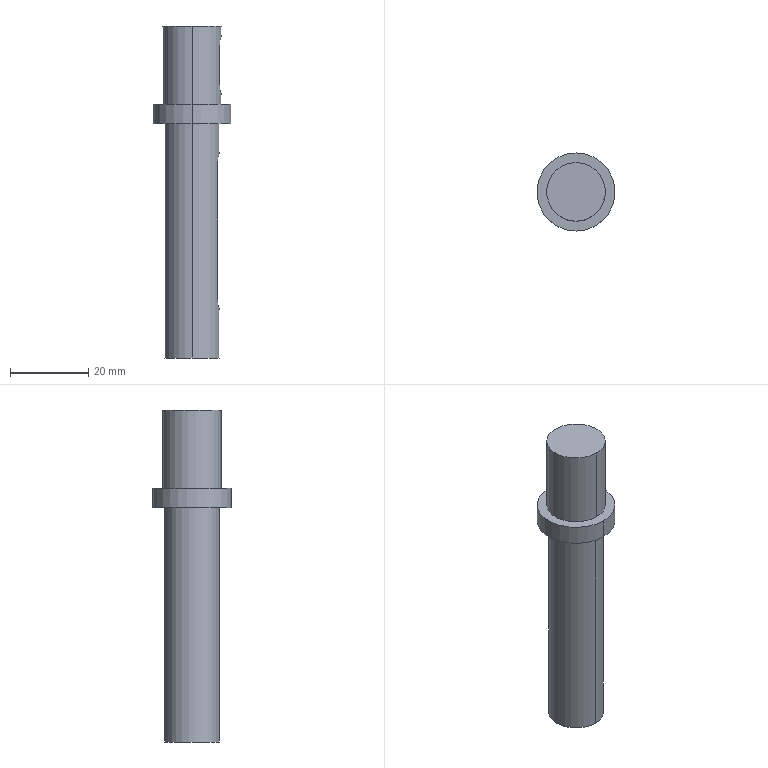Component | SolidWorks | DoubleFilmTransport-1_GearboxAxis-2 | 1 solid | 28 faces | box 20 x 20 x 85 mm | volume 13245 mm3 | cylinder 14 | plane 10 | cone 4 | commonest cylinder face diameters 5 x8 14 x2 15 x2 20 x2
build123d program:
from build123d import *

# Parameters (mm, degrees)
SKETCH1_W                    = 5
SKETCH1_H                    = 10
SKETCH2_R                    = 7.5
BOSS_EXTRUDE1_DEPTH          = 20
CUT_EXTRUDE1_REACH           = 88.724
CUT_EXTRUDE1_END_RADIUS      = 7.5
SKETCH4_R                    = 7
BOSS_EXTRUDE2_DEPTH          = 60
CUT_EXTRUDE2_REACH           = 88.724
CUT_EXTRUDE2_END_RADIUS      = 7
F_5_0_5_DIAMETER_HOLE1_D     = 5
F_5_0_5_DIAMETER_HOLE1_DEPTH = 15
F_5_0_5_DIAMETER_HOLE1_TIP   = 1.502
CHAMFER1_SIZE                = 0.525


with BuildPart() as part:
    # Sketch1 → Revolve1 (revolve)
    with BuildSketch(Plane.XY):
        with Locations((-62.5, 5)):
            Rectangle(SKETCH1_W, SKETCH1_H)
    revolve(axis=Axis((-65, 0, 0), (1, 0, 0)))

    # Sketch2 → Boss-Extrude1 (add)
    with BuildSketch(Plane.ZY.offset(65)):
        with Locations(Location((0, 0, 0), (0, 0, 270))):
            Circle(SKETCH2_R)
    extrude(amount=BOSS_EXTRUDE1_DEPTH)

    # Cut-Extrude1: up to this cylinder (the profile starts inside it)
    cut_extrude1_end = Plane(origin=(-75, 0, 0), z_dir=(1, 0, 0)) * Cylinder(CUT_EXTRUDE1_END_RADIUS, 193.448, mode=Mode.PRIVATE)
    # Sketch3 → Cut-Extrude1 (cut, up to the surface)
    with BuildSketch(Plane(origin=(0, 0, 4), x_dir=(-1, 0, 0), z_dir=(0, 0, -1)), mode=Mode.PRIVATE) as cut_extrude1_sk1:
        with BuildLine():
            Line((80, 2.5), (70, 2.5))
            ThreePointArc((70, 2.5), (67.5, 0), (70, -2.5))
            Line((70, -2.5), (80, -2.5))
            ThreePointArc((80, -2.5), (82.5, 0), (80, 2.5))
        make_face()
    cut_extrude1_tool1 = extrude(cut_extrude1_sk1.sketch, amount=-CUT_EXTRUDE1_REACH, mode=Mode.PRIVATE) & cut_extrude1_end
    add(cut_extrude1_tool1.solids().sort_by_distance((-75, 0, 4))[0], mode=Mode.SUBTRACT)

    # Sketch4 → Boss-Extrude2 (add)
    with BuildSketch(Plane(origin=(-60, 0, 0), x_dir=(0, 0, -1), z_dir=(1, 0, 0))):
        with Locations(Location((0, 0, 0), (0, 0, 90))):
            Circle(SKETCH4_R)
    extrude(amount=BOSS_EXTRUDE2_DEPTH)

    # Cut-Extrude2: up to this cylinder (the profile starts inside it)
    cut_extrude2_end = Plane(origin=(-32.5, 0, 0), z_dir=(-1, 0, 0)) * Cylinder(CUT_EXTRUDE2_END_RADIUS, 192.448, mode=Mode.PRIVATE)
    # Sketch5 → Cut-Extrude2 (cut, up to the surface)
    with BuildSketch(Plane(origin=(0, 0, 4), x_dir=(-1, 0, 0), z_dir=(0, 0, -1)), mode=Mode.PRIVATE) as cut_extrude2_sk1:
        with BuildLine():
            Line((50, 2.5), (15, 2.5))
            ThreePointArc((15, 2.5), (12.5, 0), (15, -2.5))
            Line((15, -2.5), (50, -2.5))
            ThreePointArc((50, -2.5), (52.5, 0), (50, 2.5))
        make_face()
    cut_extrude2_tool1 = extrude(cut_extrude2_sk1.sketch, amount=-CUT_EXTRUDE2_REACH, mode=Mode.PRIVATE) & cut_extrude2_end
    add(cut_extrude2_tool1.solids().sort_by_distance((-32.5, 0, 4))[0], mode=Mode.SUBTRACT)

    # 5.0 _5_ Diameter Hole1
    with Locations(Plane(origin=(0, 0, 0), x_dir=(0, 0, -1), z_dir=(1, 0, 0))):
        with Locations((0, 0)):
            Hole(F_5_0_5_DIAMETER_HOLE1_D / 2, depth=F_5_0_5_DIAMETER_HOLE1_DEPTH)
            with Locations((0, 0, -(F_5_0_5_DIAMETER_HOLE1_DEPTH + F_5_0_5_DIAMETER_HOLE1_TIP / 2))):  # 118° drill point
                Cone(0, F_5_0_5_DIAMETER_HOLE1_D / 2, F_5_0_5_DIAMETER_HOLE1_TIP, mode=Mode.SUBTRACT)

    # Chamfer1
    chamfer1_edges = [part.edges().sort_by_distance(p)[0] for p in [
        (0, 0, -2.5),
    ]]
    chamfer(chamfer1_edges, length=CHAMFER1_SIZE)


solid = part.part

# Placed as in the assembly
solid = solid.moved(Location((-374.746, 83.373, -307), (0, 90, 0)))
STEP:
#1=CARTESIAN_POINT('',(-14.655,3.282,-12.066));
#2=VERTEX_POINT('',#1);
#3=CARTESIAN_POINT('',(-14.852,3.282,-12.066));
#4=VERTEX_POINT('',#3);
#5=CARTESIAN_POINT('',(-14.754,3.282,-12.066));
#6=DIRECTION('',(-0.,-0.,-1.));
#7=DIRECTION('',(-1.,0.,0.));
#8=AXIS2_PLACEMENT_3D('',#5,#6,#7);
#9=CIRCLE('',#8,0.09843);
#10=EDGE_CURVE('',#2,#4,#9,.T.);
#11=ORIENTED_EDGE('',*,*,#10,.F.);
#12=CARTESIAN_POINT('',(-14.635,3.282,-12.087));
#13=VERTEX_POINT('',#12);
#14=CARTESIAN_POINT('',(-14.655,3.282,-12.066));
#15=DIRECTION('',(0.7071,0.,-0.7071));
#16=VECTOR('',#15,39.37);
#17=LINE('',#14,#16);
#18=EDGE_CURVE('',#2,#13,#17,.T.);
#19=ORIENTED_EDGE('',*,*,#18,.T.);
#20=CARTESIAN_POINT('',(-14.873,3.282,-12.087));
#21=VERTEX_POINT('',#20);
#22=CARTESIAN_POINT('',(-14.754,3.282,-12.087));
#23=DIRECTION('',(0.,-0.,1.));
#24=DIRECTION('',(0.,1.,0.));
#25=AXIS2_PLACEMENT_3D('',#22,#23,#24);
#26=CIRCLE('',#25,0.1191);
#27=EDGE_CURVE('',#21,#13,#26,.T.);
#28=ORIENTED_EDGE('',*,*,#27,.F.);
#29=CARTESIAN_POINT('',(-14.852,3.282,-12.066));
#30=DIRECTION('',(-0.7071,-0.,-0.7071));
#31=VECTOR('',#30,39.37);
#32=LINE('',#29,#31);
#33=EDGE_CURVE('',#4,#21,#32,.T.);
#34=ORIENTED_EDGE('',*,*,#33,.F.);
#35=EDGE_LOOP('',(#11,#19,#28,#34));
#36=FACE_OUTER_BOUND('',#35,.T.);
#37=CARTESIAN_POINT('',(-14.754,3.282,-12.066));
#38=DIRECTION('',(-0.,-0.,-1.));
#39=DIRECTION('',(-1.,0.,0.));
#40=AXIS2_PLACEMENT_3D('',#37,#38,#39);
#41=CONICAL_SURFACE('',#40,0.09843,0.7854);
#42=ADVANCED_FACE('',(#36),#41,.F.);
#43=CARTESIAN_POINT('',(-14.655,3.282,-11.496));
#44=VERTEX_POINT('',#43);
#45=CARTESIAN_POINT('',(-14.852,3.282,-11.496));
#46=VERTEX_POINT('',#45);
#47=CARTESIAN_POINT('',(-14.754,3.282,-11.496));
#48=DIRECTION('',(-0.,-0.,-1.));
#49=DIRECTION('',(-1.,0.,0.));
#50=AXIS2_PLACEMENT_3D('',#47,#48,#49);
#51=CIRCLE('',#50,0.09843);
#52=EDGE_CURVE('',#44,#46,#51,.T.);
#53=ORIENTED_EDGE('',*,*,#52,.F.);
#54=CARTESIAN_POINT('',(-14.655,3.282,-12.087));
#55=DIRECTION('',(-0.,-0.,-1.));
#56=VECTOR('',#55,39.37);
#57=LINE('',#54,#56);
#58=EDGE_CURVE('',#44,#2,#57,.T.);
#59=ORIENTED_EDGE('',*,*,#58,.T.);
#60=ORIENTED_EDGE('',*,*,#10,.T.);
#61=CARTESIAN_POINT('',(-14.852,3.282,-12.087));
#62=DIRECTION('',(-0.,-0.,-1.));
#63=VECTOR('',#62,39.37);
#64=LINE('',#61,#63);
#65=EDGE_CURVE('',#46,#4,#64,.T.);
#66=ORIENTED_EDGE('',*,*,#65,.F.);
#67=EDGE_LOOP('',(#53,#59,#60,#66));
#68=FACE_OUTER_BOUND('',#67,.T.);
#69=CARTESIAN_POINT('',(-14.754,3.282,-12.087));
#70=DIRECTION('',(-0.,-0.,-1.));
#71=DIRECTION('',(-1.,0.,0.));
#72=AXIS2_PLACEMENT_3D('',#69,#70,#71);
#73=CYLINDRICAL_SURFACE('',#72,0.09843);
#74=ADVANCED_FACE('',(#68),#73,.F.);
#75=CARTESIAN_POINT('',(-14.754,3.282,-11.437));
#76=VERTEX_POINT('',#75);
#77=CARTESIAN_POINT('',(-14.852,3.282,-11.496));
#78=DIRECTION('',(-0.8572,-0.,-0.515));
#79=VECTOR('',#78,39.37);
#80=LINE('',#77,#79);
#81=EDGE_CURVE('',#76,#46,#80,.T.);
#82=ORIENTED_EDGE('',*,*,#81,.F.);
#83=CARTESIAN_POINT('',(-14.655,3.282,-11.496));
#84=DIRECTION('',(0.8572,0.,-0.515));
#85=VECTOR('',#84,39.37);
#86=LINE('',#83,#85);
#87=EDGE_CURVE('',#76,#44,#86,.T.);
#88=ORIENTED_EDGE('',*,*,#87,.T.);
#89=ORIENTED_EDGE('',*,*,#52,.T.);
#90=EDGE_LOOP('',(#82,#88,#89));
#91=FACE_OUTER_BOUND('',#90,.T.);
#92=CARTESIAN_POINT('',(-14.754,3.282,-11.496));
#93=DIRECTION('',(-0.,-0.,-1.));
#94=DIRECTION('',(-1.,0.,0.));
#95=AXIS2_PLACEMENT_3D('',#92,#93,#94);
#96=CONICAL_SURFACE('',#95,0.09843,1.03);
#97=ADVANCED_FACE('',(#91),#96,.F.);
#98=CARTESIAN_POINT('',(-14.478,3.282,-10.02));
#99=VERTEX_POINT('',#98);
#100=CARTESIAN_POINT('',(-14.496,3.381,-10.118));
#101=VERTEX_POINT('',#100);
#102=CARTESIAN_POINT('',(-14.478,3.282,-10.02));
#103=CARTESIAN_POINT('',(-14.478,3.289,-10.02));
#104=CARTESIAN_POINT('',(-14.478,3.295,-10.02));
#105=CARTESIAN_POINT('',(-14.479,3.308,-10.023));
#106=CARTESIAN_POINT('',(-14.48,3.314,-10.025));
#107=CARTESIAN_POINT('',(-14.482,3.326,-10.03));
#108=CARTESIAN_POINT('',(-14.483,3.332,-10.033));
#109=CARTESIAN_POINT('',(-14.485,3.343,-10.04));
#110=CARTESIAN_POINT('',(-14.486,3.348,-10.044));
#111=CARTESIAN_POINT('',(-14.489,3.361,-10.058));
#112=CARTESIAN_POINT('',(-14.492,3.368,-10.068));
#113=CARTESIAN_POINT('',(-14.494,3.376,-10.086));
#114=CARTESIAN_POINT('',(-14.495,3.378,-10.092));
#115=CARTESIAN_POINT('',(-14.496,3.38,-10.105));
#116=CARTESIAN_POINT('',(-14.496,3.381,-10.112));
#117=CARTESIAN_POINT('',(-14.496,3.381,-10.118));
#118=B_SPLINE_CURVE_WITH_KNOTS('',3,(#102,#103,#104,#105,#106,#107,#108,#109,#110,#111,#112,#113,#114,#115,#116,#117),.UNSPECIFIED.,.F.,.F.,(4,2,2,2,2,2,2,4),(0.,0.0004923,0.0009846,0.001477,0.001969,0.002954,0.003446,0.003938),.UNSPECIFIED.);
#119=EDGE_CURVE('',#99,#101,#118,.T.);
#120=ORIENTED_EDGE('',*,*,#119,.F.);
#121=CARTESIAN_POINT('',(-14.596,3.282,-10.02));
#122=VERTEX_POINT('',#121);
#123=CARTESIAN_POINT('',(-14.36,3.282,-10.02));
#124=DIRECTION('',(-1.,-0.,0.));
#125=VECTOR('',#124,39.37);
#126=LINE('',#123,#125);
#127=EDGE_CURVE('',#99,#122,#126,.T.);
#128=ORIENTED_EDGE('',*,*,#127,.T.);
#129=CARTESIAN_POINT('',(-14.596,3.381,-10.118));
#130=VERTEX_POINT('',#129);
#131=CARTESIAN_POINT('',(-14.596,3.282,-10.118));
#132=DIRECTION('',(-1.,-0.,0.));
#133=DIRECTION('',(0.,0.,1.));
#134=AXIS2_PLACEMENT_3D('',#131,#132,#133);
#135=CIRCLE('',#134,0.09843);
#136=EDGE_CURVE('',#122,#130,#135,.T.);
#137=ORIENTED_EDGE('',*,*,#136,.T.);
#138=CARTESIAN_POINT('',(-14.36,3.381,-10.118));
#139=DIRECTION('',(-1.,-0.,0.));
#140=VECTOR('',#139,39.37);
#141=LINE('',#138,#140);
#142=EDGE_CURVE('',#101,#130,#141,.T.);
#143=ORIENTED_EDGE('',*,*,#142,.F.);
#144=EDGE_LOOP('',(#120,#128,#137,#143));
#145=FACE_OUTER_BOUND('',#144,.T.);
#146=CARTESIAN_POINT('',(-14.36,3.282,-10.118));
#147=DIRECTION('',(-1.,-0.,0.));
#148=DIRECTION('',(0.,0.,1.));
#149=AXIS2_PLACEMENT_3D('',#146,#147,#148);
#150=CYLINDRICAL_SURFACE('',#149,0.09843);
#151=ADVANCED_FACE('',(#145),#150,.F.);
#152=CARTESIAN_POINT('',(-14.496,3.184,-11.496));
#153=VERTEX_POINT('',#152);
#154=CARTESIAN_POINT('',(-14.496,3.184,-10.118));
#155=VERTEX_POINT('',#154);
#156=CARTESIAN_POINT('',(-14.496,3.184,-12.087));
#157=DIRECTION('',(0.,0.,1.));
#158=VECTOR('',#157,39.37);
#159=LINE('',#156,#158);
#160=EDGE_CURVE('',#153,#155,#159,.T.);
#161=ORIENTED_EDGE('',*,*,#160,.T.);
#162=CARTESIAN_POINT('',(-14.496,3.184,-10.118));
#163=CARTESIAN_POINT('',(-14.496,3.184,-10.112));
#164=CARTESIAN_POINT('',(-14.496,3.185,-10.105));
#165=CARTESIAN_POINT('',(-14.495,3.187,-10.092));
#166=CARTESIAN_POINT('',(-14.494,3.189,-10.086));
#167=CARTESIAN_POINT('',(-14.493,3.194,-10.074));
#168=CARTESIAN_POINT('',(-14.492,3.197,-10.069));
#169=CARTESIAN_POINT('',(-14.49,3.204,-10.058));
#170=CARTESIAN_POINT('',(-14.488,3.208,-10.053));
#171=CARTESIAN_POINT('',(-14.485,3.222,-10.04));
#172=CARTESIAN_POINT('',(-14.482,3.233,-10.032));
#173=CARTESIAN_POINT('',(-14.48,3.25,-10.025));
#174=CARTESIAN_POINT('',(-14.479,3.257,-10.023));
#175=CARTESIAN_POINT('',(-14.478,3.269,-10.02));
#176=CARTESIAN_POINT('',(-14.478,3.276,-10.02));
#177=CARTESIAN_POINT('',(-14.478,3.282,-10.02));
#178=B_SPLINE_CURVE_WITH_KNOTS('',3,(#162,#163,#164,#165,#166,#167,#168,#169,#170,#171,#172,#173,#174,#175,#176,#177),.UNSPECIFIED.,.F.,.F.,(4,2,2,2,2,2,2,4),(-0.003938,-0.003446,-0.002954,-0.002462,-0.001969,-0.0009846,-0.0004923,0.),.UNSPECIFIED.);
#179=EDGE_CURVE('',#155,#99,#178,.T.);
#180=ORIENTED_EDGE('',*,*,#179,.T.);
#181=ORIENTED_EDGE('',*,*,#119,.T.);
#182=CARTESIAN_POINT('',(-14.496,3.381,-11.496));
#183=VERTEX_POINT('',#182);
#184=CARTESIAN_POINT('',(-14.496,3.381,-12.087));
#185=DIRECTION('',(-0.,-0.,-1.));
#186=VECTOR('',#185,39.37);
#187=LINE('',#184,#186);
#188=EDGE_CURVE('',#101,#183,#187,.T.);
#189=ORIENTED_EDGE('',*,*,#188,.T.);
#190=CARTESIAN_POINT('',(-14.496,3.381,-11.496));
#191=CARTESIAN_POINT('',(-14.496,3.381,-11.503));
#192=CARTESIAN_POINT('',(-14.496,3.38,-11.509));
#193=CARTESIAN_POINT('',(-14.495,3.378,-11.522));
#194=CARTESIAN_POINT('',(-14.494,3.376,-11.528));
#195=CARTESIAN_POINT('',(-14.493,3.371,-11.54));
#196=CARTESIAN_POINT('',(-14.492,3.368,-11.545));
#197=CARTESIAN_POINT('',(-14.49,3.361,-11.556));
#198=CARTESIAN_POINT('',(-14.488,3.357,-11.561));
#199=CARTESIAN_POINT('',(-14.485,3.343,-11.575));
#200=CARTESIAN_POINT('',(-14.482,3.332,-11.582));
#201=CARTESIAN_POINT('',(-14.48,3.314,-11.589));
#202=CARTESIAN_POINT('',(-14.479,3.308,-11.591));
#203=CARTESIAN_POINT('',(-14.478,3.295,-11.594));
#204=CARTESIAN_POINT('',(-14.478,3.289,-11.594));
#205=CARTESIAN_POINT('',(-14.478,3.276,-11.594));
#206=CARTESIAN_POINT('',(-14.478,3.269,-11.594));
#207=CARTESIAN_POINT('',(-14.479,3.257,-11.591));
#208=CARTESIAN_POINT('',(-14.48,3.251,-11.589));
#209=CARTESIAN_POINT('',(-14.482,3.239,-11.584));
#210=CARTESIAN_POINT('',(-14.483,3.233,-11.581));
#211=CARTESIAN_POINT('',(-14.485,3.222,-11.574));
#212=CARTESIAN_POINT('',(-14.486,3.217,-11.57));
#213=CARTESIAN_POINT('',(-14.488,3.208,-11.561));
#214=CARTESIAN_POINT('',(-14.489,3.204,-11.556));
#215=CARTESIAN_POINT('',(-14.492,3.197,-11.546));
#216=CARTESIAN_POINT('',(-14.493,3.194,-11.54));
#217=CARTESIAN_POINT('',(-14.494,3.189,-11.528));
#218=CARTESIAN_POINT('',(-14.495,3.187,-11.522));
#219=CARTESIAN_POINT('',(-14.496,3.185,-11.509));
#220=CARTESIAN_POINT('',(-14.496,3.184,-11.503));
#221=CARTESIAN_POINT('',(-14.496,3.184,-11.496));
#222=B_SPLINE_CURVE_WITH_KNOTS('',3,(#190,#191,#192,#193,#194,#195,#196,#197,#198,#199,#200,#201,#202,#203,#204,#205,#206,#207,#208,#209,#210,#211,#212,#213,#214,#215,#216,#217,#218,#219,#220,#221),.UNSPECIFIED.,.F.,.F.,(4,2,2,2,2,2,2,2,2,2,2,2,2,2,2,4),(0.,0.0004924,0.0009848,0.001477,0.00197,0.002954,0.003447,0.003939,0.004432,0.004924,0.005416,0.005909,0.006401,0.006894,0.007386,0.007878),.UNSPECIFIED.);
#223=EDGE_CURVE('',#183,#153,#222,.T.);
#224=ORIENTED_EDGE('',*,*,#223,.T.);
#225=EDGE_LOOP('',(#161,#180,#181,#189,#224));
#226=FACE_BOUND('',#225,.T.);
#227=CARTESIAN_POINT('',(-14.754,3.558,-12.087));
#228=VERTEX_POINT('',#227);
#229=CARTESIAN_POINT('',(-14.754,3.007,-12.087));
#230=VERTEX_POINT('',#229);
#231=CARTESIAN_POINT('',(-14.754,3.282,-12.087));
#232=DIRECTION('',(-0.,0.,-1.));
#233=DIRECTION('',(0.,1.,0.));
#234=AXIS2_PLACEMENT_3D('',#231,#232,#233);
#235=CIRCLE('',#234,0.2756);
#236=EDGE_CURVE('',#228,#230,#235,.T.);
#237=ORIENTED_EDGE('',*,*,#236,.F.);
#238=CARTESIAN_POINT('',(-14.754,3.558,-9.724));
#239=VERTEX_POINT('',#238);
#240=CARTESIAN_POINT('',(-14.754,3.558,-12.087));
#241=DIRECTION('',(0.,-0.,1.));
#242=VECTOR('',#241,39.37);
#243=LINE('',#240,#242);
#244=EDGE_CURVE('',#228,#239,#243,.T.);
#245=ORIENTED_EDGE('',*,*,#244,.T.);
#246=CARTESIAN_POINT('',(-14.754,3.007,-9.724));
#247=VERTEX_POINT('',#246);
#248=CARTESIAN_POINT('',(-14.754,3.282,-9.724));
#249=DIRECTION('',(-0.,0.,-1.));
#250=DIRECTION('',(0.,1.,0.));
#251=AXIS2_PLACEMENT_3D('',#248,#249,#250);
#252=CIRCLE('',#251,0.2756);
#253=EDGE_CURVE('',#239,#247,#252,.T.);
#254=ORIENTED_EDGE('',*,*,#253,.T.);
#255=CARTESIAN_POINT('',(-14.754,3.007,-12.087));
#256=DIRECTION('',(0.,-0.,1.));
#257=VECTOR('',#256,39.37);
#258=LINE('',#255,#257);
#259=EDGE_CURVE('',#230,#247,#258,.T.);
#260=ORIENTED_EDGE('',*,*,#259,.F.);
#261=EDGE_LOOP('',(#237,#245,#254,#260));
#262=FACE_OUTER_BOUND('',#261,.T.);
#263=CARTESIAN_POINT('',(-14.754,3.282,-12.087));
#264=DIRECTION('',(0.,-0.,1.));
#265=DIRECTION('',(0.,-1.,0.));
#266=AXIS2_PLACEMENT_3D('',#263,#264,#265);
#267=CYLINDRICAL_SURFACE('',#266,0.2756);
#268=ADVANCED_FACE('',(#226,#262),#267,.T.);
#269=CARTESIAN_POINT('',(-14.459,3.282,-8.839));
#270=VERTEX_POINT('',#269);
#271=CARTESIAN_POINT('',(-14.475,3.381,-8.937));
#272=VERTEX_POINT('',#271);
#273=CARTESIAN_POINT('',(-14.459,3.282,-8.839));
#274=CARTESIAN_POINT('',(-14.459,3.289,-8.839));
#275=CARTESIAN_POINT('',(-14.459,3.295,-8.839));
#276=CARTESIAN_POINT('',(-14.46,3.308,-8.842));
#277=CARTESIAN_POINT('',(-14.46,3.314,-8.844));
#278=CARTESIAN_POINT('',(-14.462,3.326,-8.849));
#279=CARTESIAN_POINT('',(-14.463,3.332,-8.852));
#280=CARTESIAN_POINT('',(-14.465,3.342,-8.859));
#281=CARTESIAN_POINT('',(-14.466,3.348,-8.863));
#282=CARTESIAN_POINT('',(-14.469,3.361,-8.876));
#283=CARTESIAN_POINT('',(-14.471,3.368,-8.887));
#284=CARTESIAN_POINT('',(-14.474,3.376,-8.905));
#285=CARTESIAN_POINT('',(-14.474,3.378,-8.911));
#286=CARTESIAN_POINT('',(-14.475,3.38,-8.924));
#287=CARTESIAN_POINT('',(-14.475,3.381,-8.93));
#288=CARTESIAN_POINT('',(-14.475,3.381,-8.937));
#289=B_SPLINE_CURVE_WITH_KNOTS('',3,(#273,#274,#275,#276,#277,#278,#279,#280,#281,#282,#283,#284,#285,#286,#287,#288),.UNSPECIFIED.,.F.,.F.,(4,2,2,2,2,2,2,4),(-0.,0.0004917,0.0009835,0.001475,0.001967,0.00295,0.003442,0.003934),.UNSPECIFIED.);
#290=EDGE_CURVE('',#270,#272,#289,.T.);
#291=ORIENTED_EDGE('',*,*,#290,.F.);
#292=CARTESIAN_POINT('',(-14.596,3.282,-8.839));
#293=VERTEX_POINT('',#292);
#294=CARTESIAN_POINT('',(-14.36,3.282,-8.839));
#295=DIRECTION('',(-1.,-0.,0.));
#296=VECTOR('',#295,39.37);
#297=LINE('',#294,#296);
#298=EDGE_CURVE('',#270,#293,#297,.T.);
#299=ORIENTED_EDGE('',*,*,#298,.T.);
#300=CARTESIAN_POINT('',(-14.596,3.381,-8.937));
#301=VERTEX_POINT('',#300);
#302=CARTESIAN_POINT('',(-14.596,3.282,-8.937));
#303=DIRECTION('',(-1.,-0.,0.));
#304=DIRECTION('',(0.,0.,1.));
#305=AXIS2_PLACEMENT_3D('',#302,#303,#304);
#306=CIRCLE('',#305,0.09843);
#307=EDGE_CURVE('',#293,#301,#306,.T.);
#308=ORIENTED_EDGE('',*,*,#307,.T.);
#309=CARTESIAN_POINT('',(-14.36,3.381,-8.937));
#310=DIRECTION('',(-1.,-0.,0.));
#311=VECTOR('',#310,39.37);
#312=LINE('',#309,#311);
#313=EDGE_CURVE('',#272,#301,#312,.T.);
#314=ORIENTED_EDGE('',*,*,#313,.F.);
#315=EDGE_LOOP('',(#291,#299,#308,#314));
#316=FACE_OUTER_BOUND('',#315,.T.);
#317=CARTESIAN_POINT('',(-14.36,3.282,-8.937));
#318=DIRECTION('',(-1.,-0.,0.));
#319=DIRECTION('',(0.,0.,1.));
#320=AXIS2_PLACEMENT_3D('',#317,#318,#319);
#321=CYLINDRICAL_SURFACE('',#320,0.09843);
#322=ADVANCED_FACE('',(#316),#321,.F.);
#323=CARTESIAN_POINT('',(-14.475,3.184,-9.331));
#324=VERTEX_POINT('',#323);
#325=CARTESIAN_POINT('',(-14.475,3.184,-8.937));
#326=VERTEX_POINT('',#325);
#327=CARTESIAN_POINT('',(-14.475,3.184,-12.087));
#328=DIRECTION('',(0.,0.,1.));
#329=VECTOR('',#328,39.37);
#330=LINE('',#327,#329);
#331=EDGE_CURVE('',#324,#326,#330,.T.);
#332=ORIENTED_EDGE('',*,*,#331,.T.);
#333=CARTESIAN_POINT('',(-14.475,3.184,-8.937));
#334=CARTESIAN_POINT('',(-14.475,3.184,-8.93));
#335=CARTESIAN_POINT('',(-14.475,3.185,-8.924));
#336=CARTESIAN_POINT('',(-14.474,3.187,-8.911));
#337=CARTESIAN_POINT('',(-14.474,3.189,-8.905));
#338=CARTESIAN_POINT('',(-14.472,3.194,-8.893));
#339=CARTESIAN_POINT('',(-14.471,3.197,-8.888));
#340=CARTESIAN_POINT('',(-14.469,3.204,-8.877));
#341=CARTESIAN_POINT('',(-14.468,3.208,-8.872));
#342=CARTESIAN_POINT('',(-14.465,3.222,-8.858));
#343=CARTESIAN_POINT('',(-14.462,3.233,-8.851));
#344=CARTESIAN_POINT('',(-14.46,3.25,-8.844));
#345=CARTESIAN_POINT('',(-14.46,3.257,-8.842));
#346=CARTESIAN_POINT('',(-14.459,3.269,-8.839));
#347=CARTESIAN_POINT('',(-14.459,3.276,-8.839));
#348=CARTESIAN_POINT('',(-14.459,3.282,-8.839));
#349=B_SPLINE_CURVE_WITH_KNOTS('',3,(#333,#334,#335,#336,#337,#338,#339,#340,#341,#342,#343,#344,#345,#346,#347,#348),.UNSPECIFIED.,.F.,.F.,(4,2,2,2,2,2,2,4),(-0.003934,-0.003442,-0.00295,-0.002459,-0.001967,-0.0009835,-0.0004917,-0.),.UNSPECIFIED.);
#350=EDGE_CURVE('',#326,#270,#349,.T.);
#351=ORIENTED_EDGE('',*,*,#350,.T.);
#352=ORIENTED_EDGE('',*,*,#290,.T.);
#353=CARTESIAN_POINT('',(-14.475,3.381,-9.331));
#354=VERTEX_POINT('',#353);
#355=CARTESIAN_POINT('',(-14.475,3.381,-12.087));
#356=DIRECTION('',(-0.,-0.,-1.));
#357=VECTOR('',#356,39.37);
#358=LINE('',#355,#357);
#359=EDGE_CURVE('',#272,#354,#358,.T.);
#360=ORIENTED_EDGE('',*,*,#359,.T.);
#361=CARTESIAN_POINT('',(-14.475,3.381,-9.331));
#362=CARTESIAN_POINT('',(-14.475,3.381,-9.337));
#363=CARTESIAN_POINT('',(-14.475,3.38,-9.344));
#364=CARTESIAN_POINT('',(-14.474,3.378,-9.356));
#365=CARTESIAN_POINT('',(-14.474,3.376,-9.363));
#366=CARTESIAN_POINT('',(-14.472,3.371,-9.374));
#367=CARTESIAN_POINT('',(-14.471,3.368,-9.38));
#368=CARTESIAN_POINT('',(-14.469,3.361,-9.391));
#369=CARTESIAN_POINT('',(-14.468,3.357,-9.396));
#370=CARTESIAN_POINT('',(-14.465,3.343,-9.409));
#371=CARTESIAN_POINT('',(-14.462,3.332,-9.417));
#372=CARTESIAN_POINT('',(-14.46,3.314,-9.424));
#373=CARTESIAN_POINT('',(-14.46,3.308,-9.426));
#374=CARTESIAN_POINT('',(-14.459,3.295,-9.428));
#375=CARTESIAN_POINT('',(-14.459,3.289,-9.429));
#376=CARTESIAN_POINT('',(-14.459,3.276,-9.429));
#377=CARTESIAN_POINT('',(-14.459,3.269,-9.428));
#378=CARTESIAN_POINT('',(-14.46,3.257,-9.426));
#379=CARTESIAN_POINT('',(-14.46,3.251,-9.424));
#380=CARTESIAN_POINT('',(-14.462,3.239,-9.419));
#381=CARTESIAN_POINT('',(-14.463,3.233,-9.416));
#382=CARTESIAN_POINT('',(-14.465,3.222,-9.409));
#383=CARTESIAN_POINT('',(-14.466,3.217,-9.405));
#384=CARTESIAN_POINT('',(-14.468,3.208,-9.396));
#385=CARTESIAN_POINT('',(-14.469,3.204,-9.391));
#386=CARTESIAN_POINT('',(-14.471,3.197,-9.38));
#387=CARTESIAN_POINT('',(-14.472,3.194,-9.375));
#388=CARTESIAN_POINT('',(-14.474,3.189,-9.363));
#389=CARTESIAN_POINT('',(-14.474,3.187,-9.357));
#390=CARTESIAN_POINT('',(-14.475,3.185,-9.344));
#391=CARTESIAN_POINT('',(-14.475,3.184,-9.337));
#392=CARTESIAN_POINT('',(-14.475,3.184,-9.331));
#393=B_SPLINE_CURVE_WITH_KNOTS('',3,(#361,#362,#363,#364,#365,#366,#367,#368,#369,#370,#371,#372,#373,#374,#375,#376,#377,#378,#379,#380,#381,#382,#383,#384,#385,#386,#387,#388,#389,#390,#391,#392),.UNSPECIFIED.,.F.,.F.,(4,2,2,2,2,2,2,2,2,2,2,2,2,2,2,4),(0.,0.0004919,0.0009837,0.001476,0.001967,0.002951,0.003443,0.003935,0.004427,0.004919,0.00541,0.005902,0.006394,0.006886,0.007378,0.00787),.UNSPECIFIED.);
#394=EDGE_CURVE('',#354,#324,#393,.T.);
#395=ORIENTED_EDGE('',*,*,#394,.T.);
#396=EDGE_LOOP('',(#332,#351,#352,#360,#395));
#397=FACE_BOUND('',#396,.T.);
#398=CARTESIAN_POINT('',(-14.754,2.987,-8.74));
#399=VERTEX_POINT('',#398);
#400=CARTESIAN_POINT('',(-14.754,3.578,-8.74));
#401=VERTEX_POINT('',#400);
#402=CARTESIAN_POINT('',(-14.754,3.282,-8.74));
#403=DIRECTION('',(0.,-0.,1.));
#404=DIRECTION('',(0.,-1.,0.));
#405=AXIS2_PLACEMENT_3D('',#402,#403,#404);
#406=CIRCLE('',#405,0.2953);
#407=EDGE_CURVE('',#399,#401,#406,.T.);
#408=ORIENTED_EDGE('',*,*,#407,.F.);
#409=CARTESIAN_POINT('',(-14.754,2.987,-9.528));
#410=VERTEX_POINT('',#409);
#411=CARTESIAN_POINT('',(-14.754,2.987,-8.74));
#412=DIRECTION('',(-0.,0.,-1.));
#413=VECTOR('',#412,39.37);
#414=LINE('',#411,#413);
#415=EDGE_CURVE('',#399,#410,#414,.T.);
#416=ORIENTED_EDGE('',*,*,#415,.T.);
#417=CARTESIAN_POINT('',(-14.754,3.578,-9.528));
#418=VERTEX_POINT('',#417);
#419=CARTESIAN_POINT('',(-14.754,3.282,-9.528));
#420=DIRECTION('',(0.,-0.,1.));
#421=DIRECTION('',(0.,-1.,0.));
#422=AXIS2_PLACEMENT_3D('',#419,#420,#421);
#423=CIRCLE('',#422,0.2953);
#424=EDGE_CURVE('',#410,#418,#423,.T.);
#425=ORIENTED_EDGE('',*,*,#424,.T.);
#426=CARTESIAN_POINT('',(-14.754,3.578,-8.74));
#427=DIRECTION('',(-0.,0.,-1.));
#428=VECTOR('',#427,39.37);
#429=LINE('',#426,#428);
#430=EDGE_CURVE('',#401,#418,#429,.T.);
#431=ORIENTED_EDGE('',*,*,#430,.F.);
#432=EDGE_LOOP('',(#408,#416,#425,#431));
#433=FACE_OUTER_BOUND('',#432,.T.);
#434=CARTESIAN_POINT('',(-14.754,3.282,-8.74));
#435=DIRECTION('',(-0.,0.,-1.));
#436=DIRECTION('',(0.,1.,0.));
#437=AXIS2_PLACEMENT_3D('',#434,#435,#436);
#438=CYLINDRICAL_SURFACE('',#437,0.2953);
#439=ADVANCED_FACE('',(#397,#433),#438,.T.);
#440=CARTESIAN_POINT('',(-14.754,3.676,-9.528));
#441=VERTEX_POINT('',#440);
#442=CARTESIAN_POINT('',(-14.754,2.889,-9.528));
#443=VERTEX_POINT('',#442);
#444=CARTESIAN_POINT('',(-14.754,3.282,-9.528));
#445=DIRECTION('',(-0.,0.,-1.));
#446=DIRECTION('',(0.,1.,0.));
#447=AXIS2_PLACEMENT_3D('',#444,#445,#446);
#448=CIRCLE('',#447,0.3937);
#449=EDGE_CURVE('',#441,#443,#448,.T.);
#450=ORIENTED_EDGE('',*,*,#449,.T.);
#451=CARTESIAN_POINT('',(-14.754,2.889,-9.724));
#452=VERTEX_POINT('',#451);
#453=CARTESIAN_POINT('',(-14.754,2.889,-9.528));
#454=DIRECTION('',(-0.,0.,-1.));
#455=VECTOR('',#454,39.37);
#456=LINE('',#453,#455);
#457=EDGE_CURVE('',#443,#452,#456,.T.);
#458=ORIENTED_EDGE('',*,*,#457,.T.);
#459=CARTESIAN_POINT('',(-14.754,3.676,-9.724));
#460=VERTEX_POINT('',#459);
#461=CARTESIAN_POINT('',(-14.754,3.282,-9.724));
#462=DIRECTION('',(-0.,0.,-1.));
#463=DIRECTION('',(0.,1.,0.));
#464=AXIS2_PLACEMENT_3D('',#461,#462,#463);
#465=CIRCLE('',#464,0.3937);
#466=EDGE_CURVE('',#460,#452,#465,.T.);
#467=ORIENTED_EDGE('',*,*,#466,.F.);
#468=CARTESIAN_POINT('',(-14.754,3.676,-9.528));
#469=DIRECTION('',(-0.,0.,-1.));
#470=VECTOR('',#469,39.37);
#471=LINE('',#468,#470);
#472=EDGE_CURVE('',#441,#460,#471,.T.);
#473=ORIENTED_EDGE('',*,*,#472,.F.);
#474=EDGE_LOOP('',(#450,#458,#467,#473));
#475=FACE_OUTER_BOUND('',#474,.T.);
#476=CARTESIAN_POINT('',(-14.754,3.282,-9.528));
#477=DIRECTION('',(-0.,0.,-1.));
#478=DIRECTION('',(0.,1.,0.));
#479=AXIS2_PLACEMENT_3D('',#476,#477,#478);
#480=CYLINDRICAL_SURFACE('',#479,0.3937);
#481=ADVANCED_FACE('',(#475),#480,.T.);
#482=ORIENTED_EDGE('',*,*,#457,.F.);
#483=CARTESIAN_POINT('',(-14.754,3.282,-9.528));
#484=DIRECTION('',(-0.,0.,-1.));
#485=DIRECTION('',(0.,1.,0.));
#486=AXIS2_PLACEMENT_3D('',#483,#484,#485);
#487=CIRCLE('',#486,0.3937);
#488=EDGE_CURVE('',#443,#441,#487,.T.);
#489=ORIENTED_EDGE('',*,*,#488,.T.);
#490=ORIENTED_EDGE('',*,*,#472,.T.);
#491=CARTESIAN_POINT('',(-14.754,3.282,-9.724));
#492=DIRECTION('',(-0.,0.,-1.));
#493=DIRECTION('',(0.,1.,0.));
#494=AXIS2_PLACEMENT_3D('',#491,#492,#493);
#495=CIRCLE('',#494,0.3937);
#496=EDGE_CURVE('',#452,#460,#495,.T.);
#497=ORIENTED_EDGE('',*,*,#496,.F.);
#498=EDGE_LOOP('',(#482,#489,#490,#497));
#499=FACE_OUTER_BOUND('',#498,.T.);
#500=CARTESIAN_POINT('',(-14.754,3.282,-9.528));
#501=DIRECTION('',(-0.,0.,-1.));
#502=DIRECTION('',(0.,1.,0.));
#503=AXIS2_PLACEMENT_3D('',#500,#501,#502);
#504=CYLINDRICAL_SURFACE('',#503,0.3937);
#505=ADVANCED_FACE('',(#499),#504,.T.);
#506=CARTESIAN_POINT('',(-14.754,3.282,-9.528));
#507=DIRECTION('',(0.,-0.,1.));
#508=DIRECTION('',(0.,-1.,0.));
#509=AXIS2_PLACEMENT_3D('',#506,#507,#508);
#510=CIRCLE('',#509,0.2953);
#511=EDGE_CURVE('',#418,#410,#510,.T.);
#512=ORIENTED_EDGE('',*,*,#511,.F.);
#513=ORIENTED_EDGE('',*,*,#424,.F.);
#514=EDGE_LOOP('',(#512,#513));
#515=FACE_BOUND('',#514,.T.);
#516=ORIENTED_EDGE('',*,*,#449,.F.);
#517=ORIENTED_EDGE('',*,*,#488,.F.);
#518=EDGE_LOOP('',(#516,#517));
#519=FACE_OUTER_BOUND('',#518,.T.);
#520=CARTESIAN_POINT('',(-14.754,3.676,-9.528));
#521=DIRECTION('',(0.,-0.,1.));
#522=DIRECTION('',(0.,-1.,-0.));
#523=AXIS2_PLACEMENT_3D('',#520,#521,#522);
#524=PLANE('',#523);
#525=ADVANCED_FACE('',(#515,#519),#524,.T.);
#526=CARTESIAN_POINT('',(-14.754,3.282,-9.724));
#527=DIRECTION('',(-0.,0.,-1.));
#528=DIRECTION('',(0.,1.,0.));
#529=AXIS2_PLACEMENT_3D('',#526,#527,#528);
#530=CIRCLE('',#529,0.2756);
#531=EDGE_CURVE('',#247,#239,#530,.T.);
#532=ORIENTED_EDGE('',*,*,#531,.F.);
#533=ORIENTED_EDGE('',*,*,#253,.F.);
#534=EDGE_LOOP('',(#532,#533));
#535=FACE_BOUND('',#534,.T.);
#536=ORIENTED_EDGE('',*,*,#466,.T.);
#537=ORIENTED_EDGE('',*,*,#496,.T.);
#538=EDGE_LOOP('',(#536,#537));
#539=FACE_OUTER_BOUND('',#538,.T.);
#540=CARTESIAN_POINT('',(-14.754,3.282,-9.724));
#541=DIRECTION('',(-0.,0.,-1.));
#542=DIRECTION('',(-0.,1.,0.));
#543=AXIS2_PLACEMENT_3D('',#540,#541,#542);
#544=PLANE('',#543);
#545=ADVANCED_FACE('',(#535,#539),#544,.T.);
#546=ORIENTED_EDGE('',*,*,#415,.F.);
#547=CARTESIAN_POINT('',(-14.754,3.282,-8.74));
#548=DIRECTION('',(0.,-0.,1.));
#549=DIRECTION('',(0.,-1.,0.));
#550=AXIS2_PLACEMENT_3D('',#547,#548,#549);
#551=CIRCLE('',#550,0.2953);
#552=EDGE_CURVE('',#401,#399,#551,.T.);
#553=ORIENTED_EDGE('',*,*,#552,.F.);
#554=ORIENTED_EDGE('',*,*,#430,.T.);
#555=ORIENTED_EDGE('',*,*,#511,.T.);
#556=EDGE_LOOP('',(#546,#553,#554,#555));
#557=FACE_OUTER_BOUND('',#556,.T.);
#558=CARTESIAN_POINT('',(-14.754,3.282,-8.74));
#559=DIRECTION('',(-0.,0.,-1.));
#560=DIRECTION('',(0.,1.,0.));
#561=AXIS2_PLACEMENT_3D('',#558,#559,#560);
#562=CYLINDRICAL_SURFACE('',#561,0.2953);
#563=ADVANCED_FACE('',(#557),#562,.T.);
#564=ORIENTED_EDGE('',*,*,#552,.T.);
#565=ORIENTED_EDGE('',*,*,#407,.T.);
#566=EDGE_LOOP('',(#564,#565));
#567=FACE_OUTER_BOUND('',#566,.T.);
#568=CARTESIAN_POINT('',(-14.754,3.282,-8.74));
#569=DIRECTION('',(0.,-0.,1.));
#570=DIRECTION('',(0.,-1.,-0.));
#571=AXIS2_PLACEMENT_3D('',#568,#569,#570);
#572=PLANE('',#571);
#573=ADVANCED_FACE('',(#567),#572,.T.);
#574=ORIENTED_EDGE('',*,*,#298,.F.);
#575=ORIENTED_EDGE('',*,*,#350,.F.);
#576=CARTESIAN_POINT('',(-14.596,3.184,-8.937));
#577=VERTEX_POINT('',#576);
#578=CARTESIAN_POINT('',(-14.36,3.184,-8.937));
#579=DIRECTION('',(-1.,-0.,0.));
#580=VECTOR('',#579,39.37);
#581=LINE('',#578,#580);
#582=EDGE_CURVE('',#326,#577,#581,.T.);
#583=ORIENTED_EDGE('',*,*,#582,.T.);
#584=CARTESIAN_POINT('',(-14.596,3.282,-8.937));
#585=DIRECTION('',(-1.,-0.,0.));
#586=DIRECTION('',(0.,0.,1.));
#587=AXIS2_PLACEMENT_3D('',#584,#585,#586);
#588=CIRCLE('',#587,0.09843);
#589=EDGE_CURVE('',#577,#293,#588,.T.);
#590=ORIENTED_EDGE('',*,*,#589,.T.);
#591=EDGE_LOOP('',(#574,#575,#583,#590));
#592=FACE_OUTER_BOUND('',#591,.T.);
#593=CARTESIAN_POINT('',(-14.36,3.282,-8.937));
#594=DIRECTION('',(-1.,-0.,0.));
#595=DIRECTION('',(0.,0.,1.));
#596=AXIS2_PLACEMENT_3D('',#593,#594,#595);
#597=CYLINDRICAL_SURFACE('',#596,0.09843);
#598=ADVANCED_FACE('',(#592),#597,.F.);
#599=ORIENTED_EDGE('',*,*,#331,.F.);
#600=CARTESIAN_POINT('',(-14.596,3.184,-9.331));
#601=VERTEX_POINT('',#600);
#602=CARTESIAN_POINT('',(-14.36,3.184,-9.331));
#603=DIRECTION('',(-1.,-0.,0.));
#604=VECTOR('',#603,39.37);
#605=LINE('',#602,#604);
#606=EDGE_CURVE('',#324,#601,#605,.T.);
#607=ORIENTED_EDGE('',*,*,#606,.T.);
#608=CARTESIAN_POINT('',(-14.596,3.184,-9.331));
#609=DIRECTION('',(0.,-0.,1.));
#610=VECTOR('',#609,39.37);
#611=LINE('',#608,#610);
#612=EDGE_CURVE('',#601,#577,#611,.T.);
#613=ORIENTED_EDGE('',*,*,#612,.T.);
#614=ORIENTED_EDGE('',*,*,#582,.F.);
#615=EDGE_LOOP('',(#599,#607,#613,#614));
#616=FACE_OUTER_BOUND('',#615,.T.);
#617=CARTESIAN_POINT('',(-14.36,3.184,-9.331));
#618=DIRECTION('',(0.,-1.,-0.));
#619=DIRECTION('',(-0.,0.,-1.));
#620=AXIS2_PLACEMENT_3D('',#617,#618,#619);
#621=PLANE('',#620);
#622=ADVANCED_FACE('',(#616),#621,.F.);
#623=ORIENTED_EDGE('',*,*,#394,.F.);
#624=CARTESIAN_POINT('',(-14.596,3.381,-9.331));
#625=VERTEX_POINT('',#624);
#626=CARTESIAN_POINT('',(-14.36,3.381,-9.331));
#627=DIRECTION('',(-1.,-0.,0.));
#628=VECTOR('',#627,39.37);
#629=LINE('',#626,#628);
#630=EDGE_CURVE('',#354,#625,#629,.T.);
#631=ORIENTED_EDGE('',*,*,#630,.T.);
#632=CARTESIAN_POINT('',(-14.596,3.282,-9.331));
#633=DIRECTION('',(-1.,-0.,0.));
#634=DIRECTION('',(0.,0.,1.));
#635=AXIS2_PLACEMENT_3D('',#632,#633,#634);
#636=CIRCLE('',#635,0.09843);
#637=EDGE_CURVE('',#625,#601,#636,.T.);
#638=ORIENTED_EDGE('',*,*,#637,.T.);
#639=ORIENTED_EDGE('',*,*,#606,.F.);
#640=EDGE_LOOP('',(#623,#631,#638,#639));
#641=FACE_OUTER_BOUND('',#640,.T.);
#642=CARTESIAN_POINT('',(-14.36,3.282,-9.331));
#643=DIRECTION('',(-1.,-0.,0.));
#644=DIRECTION('',(0.,0.,1.));
#645=AXIS2_PLACEMENT_3D('',#642,#643,#644);
#646=CYLINDRICAL_SURFACE('',#645,0.09843);
#647=ADVANCED_FACE('',(#641),#646,.F.);
#648=ORIENTED_EDGE('',*,*,#359,.F.);
#649=ORIENTED_EDGE('',*,*,#313,.T.);
#650=CARTESIAN_POINT('',(-14.596,3.381,-8.937));
#651=DIRECTION('',(-0.,-0.,-1.));
#652=VECTOR('',#651,39.37);
#653=LINE('',#650,#652);
#654=EDGE_CURVE('',#301,#625,#653,.T.);
#655=ORIENTED_EDGE('',*,*,#654,.T.);
#656=ORIENTED_EDGE('',*,*,#630,.F.);
#657=EDGE_LOOP('',(#648,#649,#655,#656));
#658=FACE_OUTER_BOUND('',#657,.T.);
#659=CARTESIAN_POINT('',(-14.36,3.381,-8.937));
#660=DIRECTION('',(-0.,1.,-0.));
#661=DIRECTION('',(1.,0.,-0.));
#662=AXIS2_PLACEMENT_3D('',#659,#660,#661);
#663=PLANE('',#662);
#664=ADVANCED_FACE('',(#658),#663,.F.);
#665=ORIENTED_EDGE('',*,*,#589,.F.);
#666=ORIENTED_EDGE('',*,*,#612,.F.);
#667=ORIENTED_EDGE('',*,*,#637,.F.);
#668=ORIENTED_EDGE('',*,*,#654,.F.);
#669=ORIENTED_EDGE('',*,*,#307,.F.);
#670=EDGE_LOOP('',(#665,#666,#667,#668,#669));
#671=FACE_OUTER_BOUND('',#670,.T.);
#672=CARTESIAN_POINT('',(-14.596,3.282,-8.937));
#673=DIRECTION('',(-1.,-0.,0.));
#674=DIRECTION('',(0.,0.,1.));
#675=AXIS2_PLACEMENT_3D('',#672,#673,#674);
#676=PLANE('',#675);
#677=ADVANCED_FACE('',(#671),#676,.F.);
#678=ORIENTED_EDGE('',*,*,#244,.F.);
#679=CARTESIAN_POINT('',(-14.754,3.282,-12.087));
#680=DIRECTION('',(-0.,0.,-1.));
#681=DIRECTION('',(0.,1.,0.));
#682=AXIS2_PLACEMENT_3D('',#679,#680,#681);
#683=CIRCLE('',#682,0.2756);
#684=EDGE_CURVE('',#230,#228,#683,.T.);
#685=ORIENTED_EDGE('',*,*,#684,.F.);
#686=ORIENTED_EDGE('',*,*,#259,.T.);
#687=ORIENTED_EDGE('',*,*,#531,.T.);
#688=EDGE_LOOP('',(#678,#685,#686,#687));
#689=FACE_OUTER_BOUND('',#688,.T.);
#690=CARTESIAN_POINT('',(-14.754,3.282,-12.087));
#691=DIRECTION('',(0.,-0.,1.));
#692=DIRECTION('',(0.,-1.,0.));
#693=AXIS2_PLACEMENT_3D('',#690,#691,#692);
#694=CYLINDRICAL_SURFACE('',#693,0.2756);
#695=ADVANCED_FACE('',(#689),#694,.T.);
#696=ORIENTED_EDGE('',*,*,#27,.T.);
#697=CARTESIAN_POINT('',(-14.754,3.282,-12.087));
#698=DIRECTION('',(0.,-0.,1.));
#699=DIRECTION('',(0.,1.,0.));
#700=AXIS2_PLACEMENT_3D('',#697,#698,#699);
#701=CIRCLE('',#700,0.1191);
#702=EDGE_CURVE('',#13,#21,#701,.T.);
#703=ORIENTED_EDGE('',*,*,#702,.T.);
#704=EDGE_LOOP('',(#696,#703));
#705=FACE_BOUND('',#704,.T.);
#706=ORIENTED_EDGE('',*,*,#684,.T.);
#707=ORIENTED_EDGE('',*,*,#236,.T.);
#708=EDGE_LOOP('',(#706,#707));
#709=FACE_OUTER_BOUND('',#708,.T.);
#710=CARTESIAN_POINT('',(-14.754,3.282,-12.087));
#711=DIRECTION('',(-0.,0.,-1.));
#712=DIRECTION('',(-0.,1.,0.));
#713=AXIS2_PLACEMENT_3D('',#710,#711,#712);
#714=PLANE('',#713);
#715=ADVANCED_FACE('',(#705,#709),#714,.T.);
#716=ORIENTED_EDGE('',*,*,#127,.F.);
#717=ORIENTED_EDGE('',*,*,#179,.F.);
#718=CARTESIAN_POINT('',(-14.596,3.184,-10.118));
#719=VERTEX_POINT('',#718);
#720=CARTESIAN_POINT('',(-14.36,3.184,-10.118));
#721=DIRECTION('',(-1.,-0.,0.));
#722=VECTOR('',#721,39.37);
#723=LINE('',#720,#722);
#724=EDGE_CURVE('',#155,#719,#723,.T.);
#725=ORIENTED_EDGE('',*,*,#724,.T.);
#726=CARTESIAN_POINT('',(-14.596,3.282,-10.118));
#727=DIRECTION('',(-1.,-0.,0.));
#728=DIRECTION('',(0.,0.,1.));
#729=AXIS2_PLACEMENT_3D('',#726,#727,#728);
#730=CIRCLE('',#729,0.09843);
#731=EDGE_CURVE('',#719,#122,#730,.T.);
#732=ORIENTED_EDGE('',*,*,#731,.T.);
#733=EDGE_LOOP('',(#716,#717,#725,#732));
#734=FACE_OUTER_BOUND('',#733,.T.);
#735=CARTESIAN_POINT('',(-14.36,3.282,-10.118));
#736=DIRECTION('',(-1.,-0.,0.));
#737=DIRECTION('',(0.,0.,1.));
#738=AXIS2_PLACEMENT_3D('',#735,#736,#737);
#739=CYLINDRICAL_SURFACE('',#738,0.09843);
#740=ADVANCED_FACE('',(#734),#739,.F.);
#741=ORIENTED_EDGE('',*,*,#160,.F.);
#742=CARTESIAN_POINT('',(-14.596,3.184,-11.496));
#743=VERTEX_POINT('',#742);
#744=CARTESIAN_POINT('',(-14.36,3.184,-11.496));
#745=DIRECTION('',(-1.,-0.,0.));
#746=VECTOR('',#745,39.37);
#747=LINE('',#744,#746);
#748=EDGE_CURVE('',#153,#743,#747,.T.);
#749=ORIENTED_EDGE('',*,*,#748,.T.);
#750=CARTESIAN_POINT('',(-14.596,3.184,-11.496));
#751=DIRECTION('',(0.,0.,1.));
#752=VECTOR('',#751,39.37);
#753=LINE('',#750,#752);
#754=EDGE_CURVE('',#743,#719,#753,.T.);
#755=ORIENTED_EDGE('',*,*,#754,.T.);
#756=ORIENTED_EDGE('',*,*,#724,.F.);
#757=EDGE_LOOP('',(#741,#749,#755,#756));
#758=FACE_OUTER_BOUND('',#757,.T.);
#759=CARTESIAN_POINT('',(-14.36,3.184,-11.496));
#760=DIRECTION('',(0.,-1.,0.));
#761=DIRECTION('',(-0.,-0.,-1.));
#762=AXIS2_PLACEMENT_3D('',#759,#760,#761);
#763=PLANE('',#762);
#764=ADVANCED_FACE('',(#758),#763,.F.);
#765=ORIENTED_EDGE('',*,*,#223,.F.);
#766=CARTESIAN_POINT('',(-14.596,3.381,-11.496));
#767=VERTEX_POINT('',#766);
#768=CARTESIAN_POINT('',(-14.36,3.381,-11.496));
#769=DIRECTION('',(-1.,-0.,0.));
#770=VECTOR('',#769,39.37);
#771=LINE('',#768,#770);
#772=EDGE_CURVE('',#183,#767,#771,.T.);
#773=ORIENTED_EDGE('',*,*,#772,.T.);
#774=CARTESIAN_POINT('',(-14.596,3.282,-11.496));
#775=DIRECTION('',(-1.,-0.,0.));
#776=DIRECTION('',(0.,0.,1.));
#777=AXIS2_PLACEMENT_3D('',#774,#775,#776);
#778=CIRCLE('',#777,0.09843);
#779=EDGE_CURVE('',#767,#743,#778,.T.);
#780=ORIENTED_EDGE('',*,*,#779,.T.);
#781=ORIENTED_EDGE('',*,*,#748,.F.);
#782=EDGE_LOOP('',(#765,#773,#780,#781));
#783=FACE_OUTER_BOUND('',#782,.T.);
#784=CARTESIAN_POINT('',(-14.36,3.282,-11.496));
#785=DIRECTION('',(-1.,-0.,0.));
#786=DIRECTION('',(0.,0.,1.));
#787=AXIS2_PLACEMENT_3D('',#784,#785,#786);
#788=CYLINDRICAL_SURFACE('',#787,0.09843);
#789=ADVANCED_FACE('',(#783),#788,.F.);
#790=ORIENTED_EDGE('',*,*,#188,.F.);
#791=ORIENTED_EDGE('',*,*,#142,.T.);
#792=CARTESIAN_POINT('',(-14.596,3.381,-10.118));
#793=DIRECTION('',(-0.,-0.,-1.));
#794=VECTOR('',#793,39.37);
#795=LINE('',#792,#794);
#796=EDGE_CURVE('',#130,#767,#795,.T.);
#797=ORIENTED_EDGE('',*,*,#796,.T.);
#798=ORIENTED_EDGE('',*,*,#772,.F.);
#799=EDGE_LOOP('',(#790,#791,#797,#798));
#800=FACE_OUTER_BOUND('',#799,.T.);
#801=CARTESIAN_POINT('',(-14.36,3.381,-10.118));
#802=DIRECTION('',(-0.,1.,-0.));
#803=DIRECTION('',(0.,0.,1.));
#804=AXIS2_PLACEMENT_3D('',#801,#802,#803);
#805=PLANE('',#804);
#806=ADVANCED_FACE('',(#800),#805,.F.);
#807=ORIENTED_EDGE('',*,*,#731,.F.);
#808=ORIENTED_EDGE('',*,*,#754,.F.);
#809=ORIENTED_EDGE('',*,*,#779,.F.);
#810=ORIENTED_EDGE('',*,*,#796,.F.);
#811=ORIENTED_EDGE('',*,*,#136,.F.);
#812=EDGE_LOOP('',(#807,#808,#809,#810,#811));
#813=FACE_OUTER_BOUND('',#812,.T.);
#814=CARTESIAN_POINT('',(-14.596,3.282,-10.118));
#815=DIRECTION('',(-1.,-0.,0.));
#816=DIRECTION('',(0.,0.,1.));
#817=AXIS2_PLACEMENT_3D('',#814,#815,#816);
#818=PLANE('',#817);
#819=ADVANCED_FACE('',(#813),#818,.F.);
#820=ORIENTED_EDGE('',*,*,#87,.F.);
#821=ORIENTED_EDGE('',*,*,#81,.T.);
#822=CARTESIAN_POINT('',(-14.754,3.282,-11.496));
#823=DIRECTION('',(-0.,-0.,-1.));
#824=DIRECTION('',(-1.,0.,0.));
#825=AXIS2_PLACEMENT_3D('',#822,#823,#824);
#826=CIRCLE('',#825,0.09843);
#827=EDGE_CURVE('',#46,#44,#826,.T.);
#828=ORIENTED_EDGE('',*,*,#827,.T.);
#829=EDGE_LOOP('',(#820,#821,#828));
#830=FACE_OUTER_BOUND('',#829,.T.);
#831=CARTESIAN_POINT('',(-14.754,3.282,-11.496));
#832=DIRECTION('',(-0.,-0.,-1.));
#833=DIRECTION('',(-1.,0.,0.));
#834=AXIS2_PLACEMENT_3D('',#831,#832,#833);
#835=CONICAL_SURFACE('',#834,0.09843,1.03);
#836=ADVANCED_FACE('',(#830),#835,.F.);
#837=ORIENTED_EDGE('',*,*,#58,.F.);
#838=ORIENTED_EDGE('',*,*,#827,.F.);
#839=ORIENTED_EDGE('',*,*,#65,.T.);
#840=CARTESIAN_POINT('',(-14.754,3.282,-12.066));
#841=DIRECTION('',(-0.,-0.,-1.));
#842=DIRECTION('',(-1.,0.,0.));
#843=AXIS2_PLACEMENT_3D('',#840,#841,#842);
#844=CIRCLE('',#843,0.09843);
#845=EDGE_CURVE('',#4,#2,#844,.T.);
#846=ORIENTED_EDGE('',*,*,#845,.T.);
#847=EDGE_LOOP('',(#837,#838,#839,#846));
#848=FACE_OUTER_BOUND('',#847,.T.);
#849=CARTESIAN_POINT('',(-14.754,3.282,-12.087));
#850=DIRECTION('',(-0.,-0.,-1.));
#851=DIRECTION('',(-1.,0.,0.));
#852=AXIS2_PLACEMENT_3D('',#849,#850,#851);
#853=CYLINDRICAL_SURFACE('',#852,0.09843);
#854=ADVANCED_FACE('',(#848),#853,.F.);
#855=ORIENTED_EDGE('',*,*,#18,.F.);
#856=ORIENTED_EDGE('',*,*,#845,.F.);
#857=ORIENTED_EDGE('',*,*,#33,.T.);
#858=ORIENTED_EDGE('',*,*,#702,.F.);
#859=EDGE_LOOP('',(#855,#856,#857,#858));
#860=FACE_OUTER_BOUND('',#859,.T.);
#861=CARTESIAN_POINT('',(-14.754,3.282,-12.066));
#862=DIRECTION('',(-0.,-0.,-1.));
#863=DIRECTION('',(-1.,0.,0.));
#864=AXIS2_PLACEMENT_3D('',#861,#862,#863);
#865=CONICAL_SURFACE('',#864,0.09843,0.7854);
#866=ADVANCED_FACE('',(#860),#865,.F.);
#867=CLOSED_SHELL('',(#42,#74,#97,#151,#268,#322,#439,#481,#505,#525,#545,#563,#573,#598,#622,#647,#664,#677,#695,#715,#740,#764,#789,#806,#819,#836,#854,#866));
#868=MANIFOLD_SOLID_BREP('',#867);
#869=CARTESIAN_POINT('',(0.,0.,0.));
#870=DIRECTION('',(0.,0.,1.));
#871=DIRECTION('',(1.,0.,0.));
#872=AXIS2_PLACEMENT_3D('',#869,#870,#871);
#873=(LENGTH_UNIT()NAMED_UNIT(*)SI_UNIT($,.METRE.));
#874=LENGTH_MEASURE_WITH_UNIT(LENGTH_MEASURE(0.0254),#873);
#875=DIMENSIONAL_EXPONENTS(1.,0.,0.,0.,0.,0.,0.);
#876=(CONVERSION_BASED_UNIT('',#874)LENGTH_UNIT()NAMED_UNIT(#875));
#877=UNCERTAINTY_MEASURE_WITH_UNIT(LENGTH_MEASURE(0.00001),#876,'','');
#878=(NAMED_UNIT(*)PLANE_ANGLE_UNIT()SI_UNIT($,.RADIAN.));
#879=(NAMED_UNIT(*)SI_UNIT($,.STERADIAN.)SOLID_ANGLE_UNIT());
#880=(GEOMETRIC_REPRESENTATION_CONTEXT(3)GLOBAL_UNCERTAINTY_ASSIGNED_CONTEXT((#877))GLOBAL_UNIT_ASSIGNED_CONTEXT((#876,#878,#879))REPRESENTATION_CONTEXT('',''));
#881=ADVANCED_BREP_SHAPE_REPRESENTATION('',(#868,#872),#880);
#882=COLOUR_RGB('',0.7922,0.8196,0.9333);
#883=FILL_AREA_STYLE_COLOUR('',#882);
#884=FILL_AREA_STYLE('',(#883));
#885=SURFACE_STYLE_FILL_AREA(#884);
#886=SURFACE_SIDE_STYLE('',(#885));
#887=SURFACE_STYLE_USAGE(.BOTH.,#886);
#888=PRESENTATION_STYLE_ASSIGNMENT((#887));
#889=STYLED_ITEM('',(#888),#868);
#890=PRESENTATION_LAYER_ASSIGNMENT('','',(#889));
#891=(LENGTH_UNIT()NAMED_UNIT(*)SI_UNIT($,.METRE.));
#892=LENGTH_MEASURE_WITH_UNIT(LENGTH_MEASURE(0.0254),#891);
#893=DIMENSIONAL_EXPONENTS(1.,0.,0.,0.,0.,0.,0.);
#894=(CONVERSION_BASED_UNIT('',#892)LENGTH_UNIT()NAMED_UNIT(#893));
#895=UNCERTAINTY_MEASURE_WITH_UNIT(LENGTH_MEASURE(0.00001),#894,'','');
#896=(NAMED_UNIT(*)PLANE_ANGLE_UNIT()SI_UNIT($,.RADIAN.));
#897=(NAMED_UNIT(*)SI_UNIT($,.STERADIAN.)SOLID_ANGLE_UNIT());
#898=(GEOMETRIC_REPRESENTATION_CONTEXT(3)GLOBAL_UNCERTAINTY_ASSIGNED_CONTEXT((#895))GLOBAL_UNIT_ASSIGNED_CONTEXT((#894,#896,#897))REPRESENTATION_CONTEXT('',''));
#899=MECHANICAL_DESIGN_GEOMETRIC_PRESENTATION_REPRESENTATION('',(#889),#898);